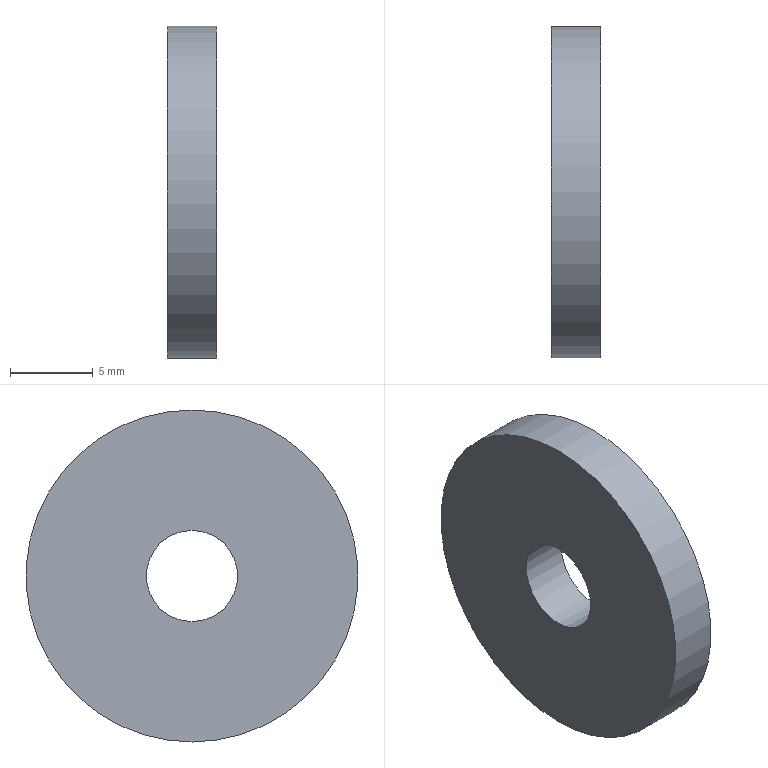Component | NX | CIRCLIP_3 | 1 solid | 4 faces | box 3 x 20 x 20 mm | volume 871 mm3 | cylinder 2 | plane 2 | commonest cylinder face diameters 20 x1 5.5 x1
STEP:
#1=CARTESIAN_POINT('',(0.,0.,0.));
#2=DIRECTION('',(0.,0.,1.));
#3=DIRECTION('',(1.,0.,0.));
#4=AXIS2_PLACEMENT_3D('',#1,#2,#3);
#5=CARTESIAN_POINT('',(70.,87.,-0.));
#6=VERTEX_POINT('',#5);
#7=CARTESIAN_POINT('',(70.,87.,10.));
#8=DIRECTION('',(1.,0.,0.));
#9=DIRECTION('',(0.,0.,-1.));
#10=AXIS2_PLACEMENT_3D('',#7,#8,#9);
#11=CIRCLE('',#10,10.);
#12=CARTESIAN_POINT('',(70.,87.,10.));
#13=DIRECTION('',(-1.,0.,0.));
#14=DIRECTION('',(0.,0.,1.));
#15=AXIS2_PLACEMENT_3D('',#12,#13,#14);
#16=CYLINDRICAL_SURFACE('',#15,10.);
#17=CARTESIAN_POINT('',(9.425,0.));
#18=DIRECTION('',(-1.,0.));
#19=VECTOR('',#18,1.);
#20=LINE('',#17,#19);
#21=(GEOMETRIC_REPRESENTATION_CONTEXT(2)PARAMETRIC_REPRESENTATION_CONTEXT()REPRESENTATION_CONTEXT('',''));
#22=DEFINITIONAL_REPRESENTATION('',(#20),#21);
#23=PCURVE('',#16,#22);
#24=CARTESIAN_POINT('',(70.,87.,10.));
#25=DIRECTION('',(1.,0.,0.));
#26=DIRECTION('',(0.,0.,-1.));
#27=AXIS2_PLACEMENT_3D('',#24,#25,#26);
#28=PLANE('',#27);
#29=CARTESIAN_POINT('',(0.,0.));
#30=DIRECTION('',(1.,0.));
#31=AXIS2_PLACEMENT_2D('',#29,#30);
#32=CIRCLE('',#31,10.);
#33=(GEOMETRIC_REPRESENTATION_CONTEXT(2)PARAMETRIC_REPRESENTATION_CONTEXT()REPRESENTATION_CONTEXT('',''));
#34=DEFINITIONAL_REPRESENTATION('',(#32),#33);
#35=PCURVE('',#28,#34);
#36=SURFACE_CURVE('',#11,(#23,#35),.PCURVE_S1.);
#37=EDGE_CURVE('',#6,#6,#36,.T.);
#38=ORIENTED_EDGE('',*,*,#37,.F.);
#39=CARTESIAN_POINT('',(67.,87.,-0.));
#40=VERTEX_POINT('',#39);
#41=CARTESIAN_POINT('',(70.,87.,0.));
#42=CARTESIAN_POINT('',(67.,87.,0.));
#43=B_SPLINE_CURVE_WITH_KNOTS('',1,(#41,#42),.UNSPECIFIED.,.F.,.F.,(2,2),(0.,3.),.PIECEWISE_BEZIER_KNOTS.);
#44=CARTESIAN_POINT('',(9.425,0.));
#45=DIRECTION('',(0.,1.));
#46=VECTOR('',#45,1.);
#47=LINE('',#44,#46);
#48=(GEOMETRIC_REPRESENTATION_CONTEXT(2)PARAMETRIC_REPRESENTATION_CONTEXT()REPRESENTATION_CONTEXT('',''));
#49=DEFINITIONAL_REPRESENTATION('',(#47),#48);
#50=PCURVE('',#16,#49);
#51=CARTESIAN_POINT('',(3.142,0.));
#52=DIRECTION('',(0.,1.));
#53=VECTOR('',#52,1.);
#54=LINE('',#51,#53);
#55=(GEOMETRIC_REPRESENTATION_CONTEXT(2)PARAMETRIC_REPRESENTATION_CONTEXT()REPRESENTATION_CONTEXT('',''));
#56=DEFINITIONAL_REPRESENTATION('',(#54),#55);
#57=PCURVE('',#16,#56);
#58=SEAM_CURVE('',#43,(#50,#57),.PCURVE_S1.);
#59=EDGE_CURVE('',#6,#40,#58,.T.);
#60=ORIENTED_EDGE('',*,*,#59,.T.);
#61=CARTESIAN_POINT('',(67.,87.,10.));
#62=DIRECTION('',(1.,0.,0.));
#63=DIRECTION('',(0.,0.,-1.));
#64=AXIS2_PLACEMENT_3D('',#61,#62,#63);
#65=CIRCLE('',#64,10.);
#66=CARTESIAN_POINT('',(9.425,3.));
#67=DIRECTION('',(-1.,0.));
#68=VECTOR('',#67,1.);
#69=LINE('',#66,#68);
#70=(GEOMETRIC_REPRESENTATION_CONTEXT(2)PARAMETRIC_REPRESENTATION_CONTEXT()REPRESENTATION_CONTEXT('',''));
#71=DEFINITIONAL_REPRESENTATION('',(#69),#70);
#72=PCURVE('',#16,#71);
#73=CARTESIAN_POINT('',(67.,87.,10.));
#74=DIRECTION('',(1.,0.,0.));
#75=DIRECTION('',(0.,0.,-1.));
#76=AXIS2_PLACEMENT_3D('',#73,#74,#75);
#77=PLANE('',#76);
#78=CARTESIAN_POINT('',(0.,0.));
#79=DIRECTION('',(1.,0.));
#80=AXIS2_PLACEMENT_2D('',#78,#79);
#81=CIRCLE('',#80,10.);
#82=(GEOMETRIC_REPRESENTATION_CONTEXT(2)PARAMETRIC_REPRESENTATION_CONTEXT()REPRESENTATION_CONTEXT('',''));
#83=DEFINITIONAL_REPRESENTATION('',(#81),#82);
#84=PCURVE('',#77,#83);
#85=SURFACE_CURVE('',#65,(#72,#84),.PCURVE_S1.);
#86=EDGE_CURVE('',#40,#40,#85,.T.);
#87=ORIENTED_EDGE('',*,*,#86,.T.);
#88=ORIENTED_EDGE('',*,*,#59,.F.);
#89=EDGE_LOOP('',(#38,#60,#87,#88));
#90=FACE_BOUND('',#89,.T.);
#91=ADVANCED_FACE('',(#90),#16,.T.);
#92=CARTESIAN_POINT('',(70.,87.,7.25));
#93=VERTEX_POINT('',#92);
#94=CARTESIAN_POINT('',(70.,87.,10.));
#95=DIRECTION('',(1.,0.,0.));
#96=DIRECTION('',(0.,0.,-1.));
#97=AXIS2_PLACEMENT_3D('',#94,#95,#96);
#98=CIRCLE('',#97,2.75);
#99=CARTESIAN_POINT('',(70.,87.,10.));
#100=DIRECTION('',(-1.,0.,0.));
#101=DIRECTION('',(0.,0.,1.));
#102=AXIS2_PLACEMENT_3D('',#99,#100,#101);
#103=CYLINDRICAL_SURFACE('',#102,2.75);
#104=CARTESIAN_POINT('',(9.425,0.));
#105=DIRECTION('',(-1.,0.));
#106=VECTOR('',#105,1.);
#107=LINE('',#104,#106);
#108=(GEOMETRIC_REPRESENTATION_CONTEXT(2)PARAMETRIC_REPRESENTATION_CONTEXT()REPRESENTATION_CONTEXT('',''));
#109=DEFINITIONAL_REPRESENTATION('',(#107),#108);
#110=PCURVE('',#103,#109);
#111=CARTESIAN_POINT('',(0.,0.));
#112=DIRECTION('',(1.,0.));
#113=AXIS2_PLACEMENT_2D('',#111,#112);
#114=CIRCLE('',#113,2.75);
#115=(GEOMETRIC_REPRESENTATION_CONTEXT(2)PARAMETRIC_REPRESENTATION_CONTEXT()REPRESENTATION_CONTEXT('',''));
#116=DEFINITIONAL_REPRESENTATION('',(#114),#115);
#117=PCURVE('',#28,#116);
#118=SURFACE_CURVE('',#98,(#110,#117),.PCURVE_S1.);
#119=EDGE_CURVE('',#93,#93,#118,.T.);
#120=ORIENTED_EDGE('',*,*,#119,.F.);
#121=CARTESIAN_POINT('',(67.,87.,7.25));
#122=VERTEX_POINT('',#121);
#123=CARTESIAN_POINT('',(70.,87.,7.25));
#124=CARTESIAN_POINT('',(67.,87.,7.25));
#125=B_SPLINE_CURVE_WITH_KNOTS('',1,(#123,#124),.UNSPECIFIED.,.F.,.F.,(2,2),(0.,3.),.PIECEWISE_BEZIER_KNOTS.);
#126=CARTESIAN_POINT('',(9.425,0.));
#127=DIRECTION('',(0.,1.));
#128=VECTOR('',#127,1.);
#129=LINE('',#126,#128);
#130=(GEOMETRIC_REPRESENTATION_CONTEXT(2)PARAMETRIC_REPRESENTATION_CONTEXT()REPRESENTATION_CONTEXT('',''));
#131=DEFINITIONAL_REPRESENTATION('',(#129),#130);
#132=PCURVE('',#103,#131);
#133=CARTESIAN_POINT('',(3.142,0.));
#134=DIRECTION('',(0.,1.));
#135=VECTOR('',#134,1.);
#136=LINE('',#133,#135);
#137=(GEOMETRIC_REPRESENTATION_CONTEXT(2)PARAMETRIC_REPRESENTATION_CONTEXT()REPRESENTATION_CONTEXT('',''));
#138=DEFINITIONAL_REPRESENTATION('',(#136),#137);
#139=PCURVE('',#103,#138);
#140=SEAM_CURVE('',#125,(#132,#139),.PCURVE_S1.);
#141=EDGE_CURVE('',#93,#122,#140,.T.);
#142=ORIENTED_EDGE('',*,*,#141,.T.);
#143=CARTESIAN_POINT('',(67.,87.,10.));
#144=DIRECTION('',(1.,0.,0.));
#145=DIRECTION('',(0.,0.,-1.));
#146=AXIS2_PLACEMENT_3D('',#143,#144,#145);
#147=CIRCLE('',#146,2.75);
#148=CARTESIAN_POINT('',(9.425,3.));
#149=DIRECTION('',(-1.,0.));
#150=VECTOR('',#149,1.);
#151=LINE('',#148,#150);
#152=(GEOMETRIC_REPRESENTATION_CONTEXT(2)PARAMETRIC_REPRESENTATION_CONTEXT()REPRESENTATION_CONTEXT('',''));
#153=DEFINITIONAL_REPRESENTATION('',(#151),#152);
#154=PCURVE('',#103,#153);
#155=CARTESIAN_POINT('',(0.,0.));
#156=DIRECTION('',(1.,0.));
#157=AXIS2_PLACEMENT_2D('',#155,#156);
#158=CIRCLE('',#157,2.75);
#159=(GEOMETRIC_REPRESENTATION_CONTEXT(2)PARAMETRIC_REPRESENTATION_CONTEXT()REPRESENTATION_CONTEXT('',''));
#160=DEFINITIONAL_REPRESENTATION('',(#158),#159);
#161=PCURVE('',#77,#160);
#162=SURFACE_CURVE('',#147,(#154,#161),.PCURVE_S1.);
#163=EDGE_CURVE('',#122,#122,#162,.T.);
#164=ORIENTED_EDGE('',*,*,#163,.T.);
#165=ORIENTED_EDGE('',*,*,#141,.F.);
#166=EDGE_LOOP('',(#120,#142,#164,#165));
#167=FACE_BOUND('',#166,.F.);
#168=ADVANCED_FACE('',(#167),#103,.F.);
#169=ORIENTED_EDGE('',*,*,#37,.T.);
#170=EDGE_LOOP('',(#169));
#171=FACE_BOUND('',#170,.T.);
#172=ORIENTED_EDGE('',*,*,#119,.F.);
#173=EDGE_LOOP('',(#172));
#174=FACE_BOUND('',#173,.T.);
#175=ADVANCED_FACE('',(#171,#174),#28,.T.);
#176=ORIENTED_EDGE('',*,*,#86,.F.);
#177=EDGE_LOOP('',(#176));
#178=FACE_BOUND('',#177,.T.);
#179=ORIENTED_EDGE('',*,*,#163,.T.);
#180=EDGE_LOOP('',(#179));
#181=FACE_BOUND('',#180,.T.);
#182=ADVANCED_FACE('',(#178,#181),#77,.F.);
#183=CLOSED_SHELL('',(#91,#168,#175,#182));
#184=MANIFOLD_SOLID_BREP('',#183);
#185=(LENGTH_UNIT()NAMED_UNIT(*)SI_UNIT(.MILLI.,.METRE.));
#186=UNCERTAINTY_MEASURE_WITH_UNIT(LENGTH_MEASURE(0.00001),#185,'','');
#187=(NAMED_UNIT(*)PLANE_ANGLE_UNIT()SI_UNIT($,.RADIAN.));
#188=(NAMED_UNIT(*)SI_UNIT($,.STERADIAN.)SOLID_ANGLE_UNIT());
#189=(GEOMETRIC_REPRESENTATION_CONTEXT(3)GLOBAL_UNCERTAINTY_ASSIGNED_CONTEXT((#186))GLOBAL_UNIT_ASSIGNED_CONTEXT((#185,#187,#188))REPRESENTATION_CONTEXT('',''));
#190=ADVANCED_BREP_SHAPE_REPRESENTATION('',(#4,#184),#189);